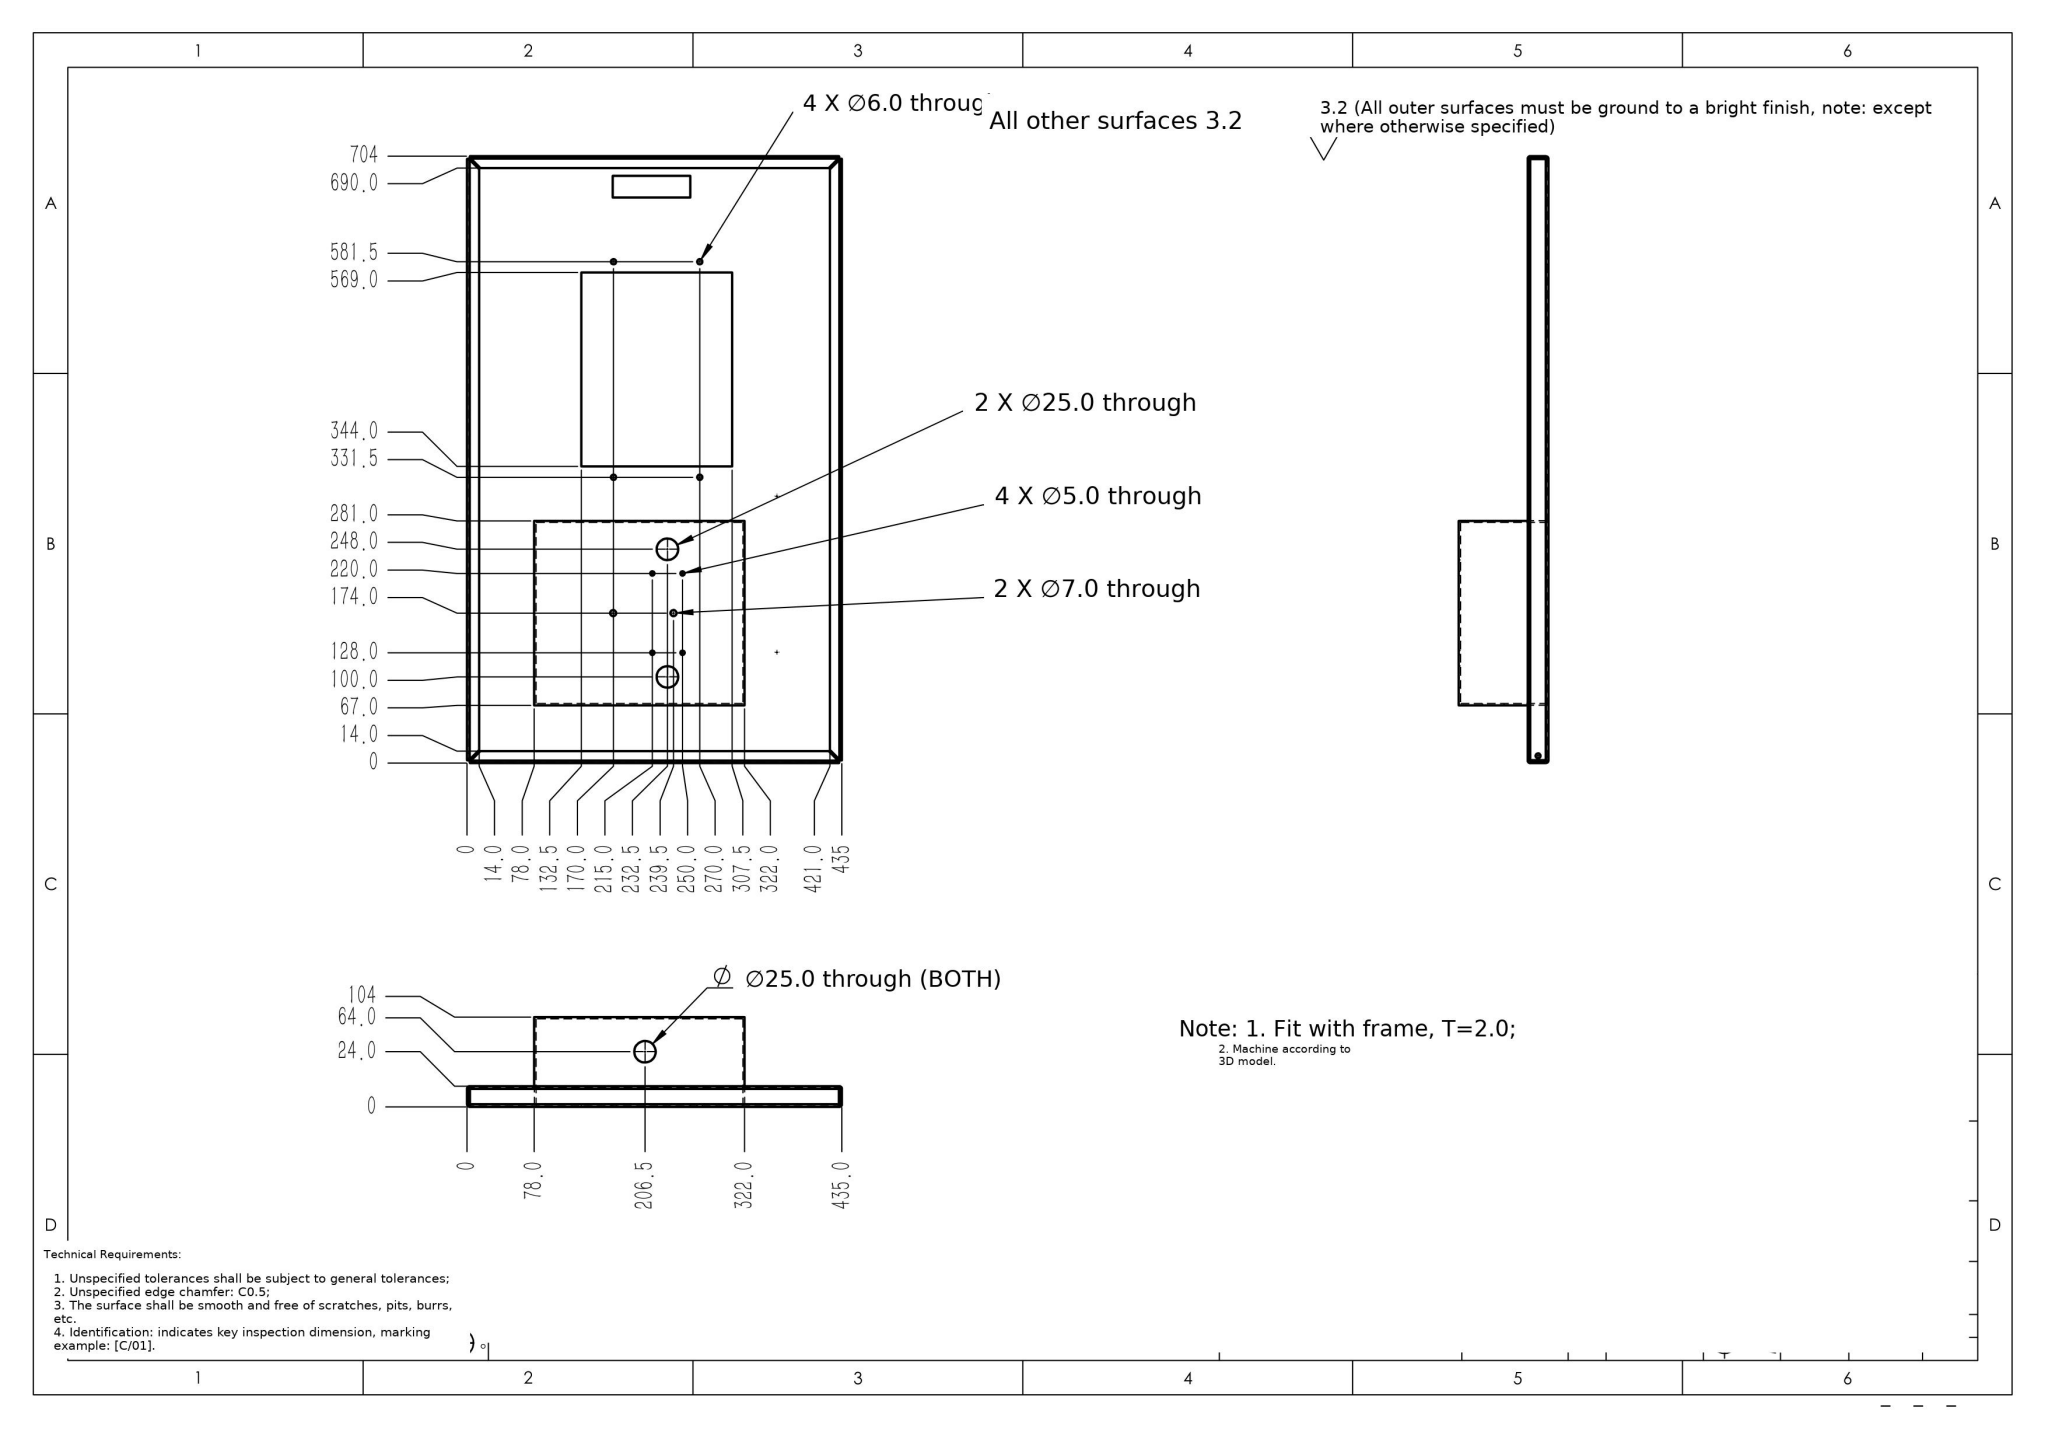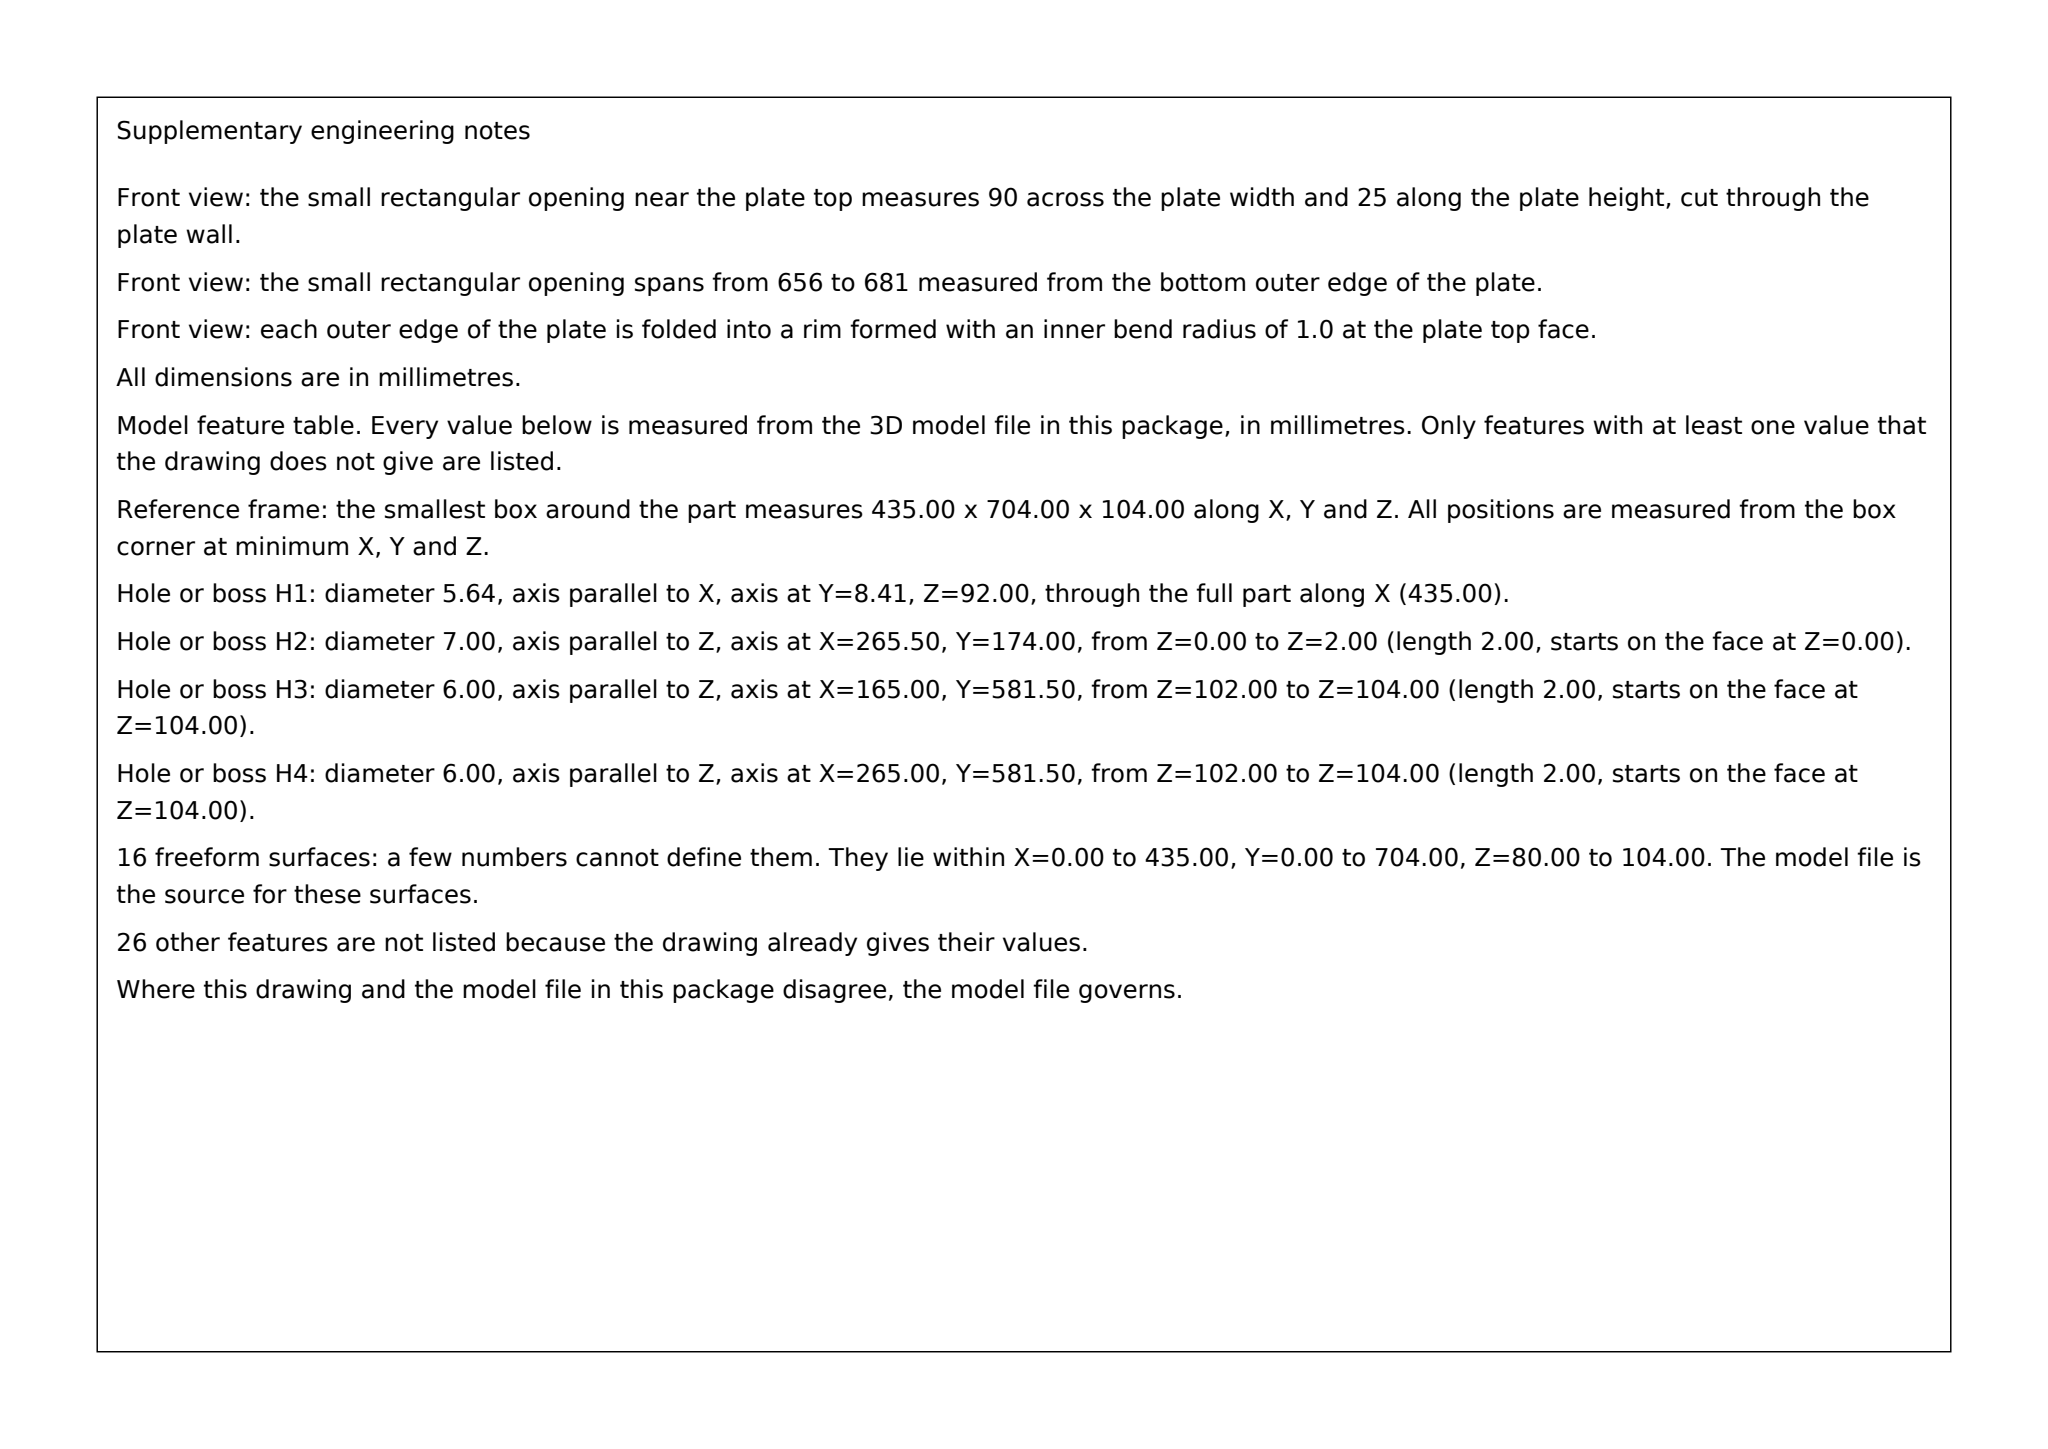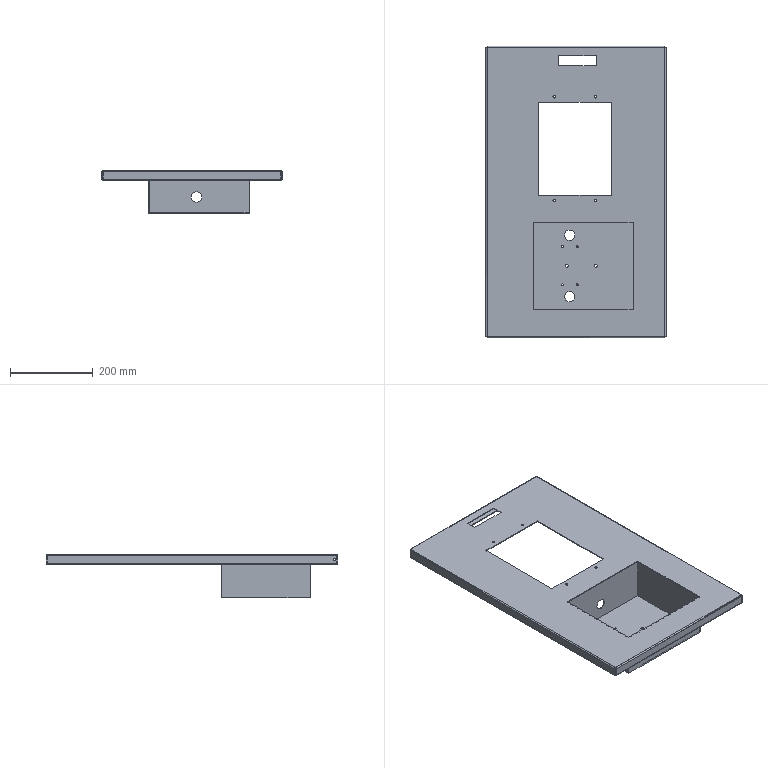Part | SolidWorks | mm | 1 solid | 124 faces | box 435 x 704 x 104 mm | volume 853967 mm3 | plane 60 | cylinder 48 | spline 16 | commonest cylinder face diameters 6 x16 25 x8 5 x8 2 x8 7 x4 5.632 x4
Drawing notes:
4X Ø6.0 THRU AT X165.0/X265.0, Y331.5/Y581.5 | from the solid: cyl dia6.0 axis z at (165.02,331.52),(165.02,581.52),(265.02,331.52),(265.02,581.52), len 2.0
TOP SLOT 90.0 X 25.0 THRU, X176.0 TO X266.0, Y656.0 TO Y681.0 | from the solid: x planes 176.02 & 266.02 (90 wide), y planes 656.02 & 681.02 (25 high), thru T=2.0
RAISED BOX/BOSS X EXTENTS: X115.0 TO X355.0 FROM X0 DATUM (Y67.0 TO Y281.0 AS SHOWN). | from the solid: axis_planes x 115.02 (2) and x 355.02 (2); y 67.02 / y 281.02
RAISED BOX/BOSS Z FACES: Z80.0 AND Z82.0 (LOWER/INNER), Z102.0 AND Z104.0 (TOP), MEASURED FROM BASE PLATE BOTTOM Z0; BOX TOP WALL 2.0 THK. | from the solid: axis_planes z 80.0 (4), z 82.0 (4), z 102.0, z 104.0
RAISED BOX INTERNAL STEP FACES: X127.5 AND X302.5; Y69.0 AND Y279.0 FROM X0/Y0 DATUM (12.5 WALL IN X, 2.0 WALL IN Y). | from the solid: axis_planes x 127.52, x 302.52; y 69.02 (2), y 279.02 (2)
4X Ø5.0 THRU (2.0 DEEP) AT X185.0 AND X220.0, Y128.0 AND Y220.0 FROM X0/Y0 DATUM. | from the solid: cylinders dia 5.0 axis z at (185.02,128.02),(185.02,220.02),(220.02,128.02),(220.02,220.02), length 2.0
2X Ø7.0 THRU (2.0 DEEP) AT X195.5 AND X265.5, Y174.0 FROM X0/Y0 DATUM. | from the solid: cylinders dia 7.0 axis z at (195.52,174.02) and (265.52,174.02), length 2.0
2X Ø25.0 THRU BASE PLATE AT X202.5, Y100.0 AND Y248.0 FROM X0/Y0 DATUM. | from the solid: cylinders dia 25.0 axis z at (202.52,100.02) and (202.52,248.02), length 2.0
PERIMETER FRAME TUBE: Ø6.0 OD X Ø2.0 ID (2.0 WALL), 2 TUBES PER SIDE AT Z83.0 AND Z101.0, AXES INSET 3.0 FROM EACH OUTER EDGE (X3.0 / X432.0, Y3.0 / Y701.0). | from the solid: cylinders dia 6.0 and 2.0, axes x/y at offsets 3.02 and 432.02 / 701.02, z 83.0 and 101.0
2X Ø5.63 THRU FRAME WALL (2.0 DEEP), AXIS PARALLEL TO X, AT Y8.4, Z92.0 FROM Y0/Z0 DATUM. | from the solid: cylinders: ["hole/bore",5.63,"x",[null,8.4,92.0],from 0.0 to 2.0, count 1] and ["hole/bore",5.63,"x",[null,8.4,92.0],from 433.0 to 435.0, count 1] = only 2 such holes, each 2.0 deep, at Y8.4 / Z92.0